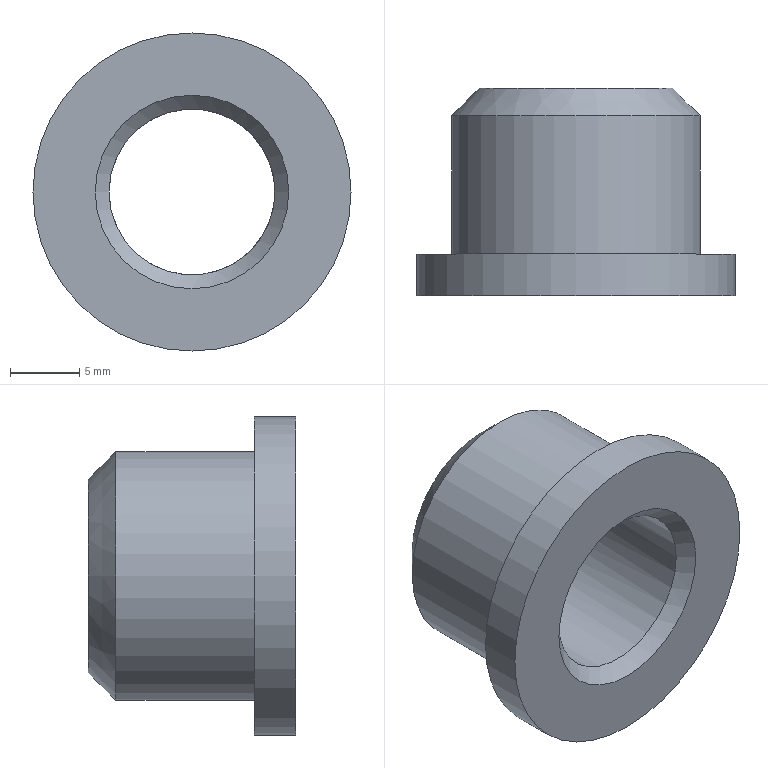Component | NX | LOCATING_BUSH | 1 solid | 8 faces | box 23 x 15 x 23 mm | volume 2479 mm3 | cylinder 3 | plane 3 | cone 2 | commonest cylinder face diameters 12 x1 18 x1 23 x1
STEP:
#1=CARTESIAN_POINT('',(0.,0.,0.));
#2=DIRECTION('',(0.,0.,1.));
#3=DIRECTION('',(1.,0.,0.));
#4=AXIS2_PLACEMENT_3D('',#1,#2,#3);
#5=CARTESIAN_POINT('',(-23.,5.,45.));
#6=VERTEX_POINT('',#5);
#7=CARTESIAN_POINT('',(-11.,5.,45.));
#8=VERTEX_POINT('',#7);
#9=CARTESIAN_POINT('',(-17.,5.,45.));
#10=DIRECTION('',(0.,-1.,0.));
#11=DIRECTION('',(1.,0.,0.));
#12=AXIS2_PLACEMENT_3D('',#9,#10,#11);
#13=CIRCLE('',#12,6.);
#14=CARTESIAN_POINT('',(-17.,19.,45.));
#15=DIRECTION('',(0.,1.,0.));
#16=DIRECTION('',(-1.,0.,0.));
#17=AXIS2_PLACEMENT_3D('',#14,#15,#16);
#18=CYLINDRICAL_SURFACE('',#17,6.);
#19=CARTESIAN_POINT('',(9.425,-14.));
#20=DIRECTION('',(-1.,0.));
#21=VECTOR('',#20,1.);
#22=LINE('',#19,#21);
#23=(GEOMETRIC_REPRESENTATION_CONTEXT(2)PARAMETRIC_REPRESENTATION_CONTEXT()REPRESENTATION_CONTEXT('',''));
#24=DEFINITIONAL_REPRESENTATION('',(#22),#23);
#25=PCURVE('',#18,#24);
#26=CARTESIAN_POINT('',(-17.,4.,45.));
#27=DIRECTION('',(0.,-1.,0.));
#28=DIRECTION('',(1.,0.,0.));
#29=AXIS2_PLACEMENT_3D('',#26,#27,#28);
#30=CONICAL_SURFACE('',#29,7.,0.7854);
#31=CARTESIAN_POINT('',(0.,-1.));
#32=DIRECTION('',(1.,0.));
#33=VECTOR('',#32,1.);
#34=LINE('',#31,#33);
#35=(GEOMETRIC_REPRESENTATION_CONTEXT(2)PARAMETRIC_REPRESENTATION_CONTEXT()REPRESENTATION_CONTEXT('',''));
#36=DEFINITIONAL_REPRESENTATION('',(#34),#35);
#37=PCURVE('',#30,#36);
#38=SURFACE_CURVE('',#13,(#25,#37),.PCURVE_S1.);
#39=EDGE_CURVE('',#6,#8,#38,.T.);
#40=ORIENTED_EDGE('',*,*,#39,.F.);
#41=CARTESIAN_POINT('',(-23.,19.,45.));
#42=VERTEX_POINT('',#41);
#43=CARTESIAN_POINT('',(-23.,5.,45.));
#44=CARTESIAN_POINT('',(-23.,19.,45.));
#45=B_SPLINE_CURVE_WITH_KNOTS('',1,(#43,#44),.UNSPECIFIED.,.F.,.F.,(2,2),(-14.,0.),.PIECEWISE_BEZIER_KNOTS.);
#46=CARTESIAN_POINT('',(6.283,0.));
#47=DIRECTION('',(0.,1.));
#48=VECTOR('',#47,1.);
#49=LINE('',#46,#48);
#50=(GEOMETRIC_REPRESENTATION_CONTEXT(2)PARAMETRIC_REPRESENTATION_CONTEXT()REPRESENTATION_CONTEXT('',''));
#51=DEFINITIONAL_REPRESENTATION('',(#49),#50);
#52=PCURVE('',#18,#51);
#53=CARTESIAN_POINT('',(0.,0.));
#54=DIRECTION('',(0.,1.));
#55=VECTOR('',#54,1.);
#56=LINE('',#53,#55);
#57=(GEOMETRIC_REPRESENTATION_CONTEXT(2)PARAMETRIC_REPRESENTATION_CONTEXT()REPRESENTATION_CONTEXT('',''));
#58=DEFINITIONAL_REPRESENTATION('',(#56),#57);
#59=PCURVE('',#18,#58);
#60=SEAM_CURVE('',#45,(#52,#59),.PCURVE_S1.);
#61=EDGE_CURVE('',#6,#42,#60,.T.);
#62=ORIENTED_EDGE('',*,*,#61,.T.);
#63=CARTESIAN_POINT('',(-17.,19.,45.));
#64=DIRECTION('',(0.,1.,0.));
#65=DIRECTION('',(-1.,0.,0.));
#66=AXIS2_PLACEMENT_3D('',#63,#64,#65);
#67=CIRCLE('',#66,6.);
#68=CARTESIAN_POINT('',(0.,0.));
#69=DIRECTION('',(1.,0.));
#70=VECTOR('',#69,1.);
#71=LINE('',#68,#70);
#72=(GEOMETRIC_REPRESENTATION_CONTEXT(2)PARAMETRIC_REPRESENTATION_CONTEXT()REPRESENTATION_CONTEXT('',''));
#73=DEFINITIONAL_REPRESENTATION('',(#71),#72);
#74=PCURVE('',#18,#73);
#75=CARTESIAN_POINT('',(-11.,19.,45.));
#76=DIRECTION('',(0.,1.,0.));
#77=DIRECTION('',(-1.,0.,0.));
#78=AXIS2_PLACEMENT_3D('',#75,#76,#77);
#79=PLANE('',#78);
#80=CARTESIAN_POINT('',(6.,0.));
#81=DIRECTION('',(1.,0.));
#82=AXIS2_PLACEMENT_2D('',#80,#81);
#83=CIRCLE('',#82,6.);
#84=(GEOMETRIC_REPRESENTATION_CONTEXT(2)PARAMETRIC_REPRESENTATION_CONTEXT()REPRESENTATION_CONTEXT('',''));
#85=DEFINITIONAL_REPRESENTATION('',(#83),#84);
#86=PCURVE('',#79,#85);
#87=SURFACE_CURVE('',#67,(#74,#86),.PCURVE_S1.);
#88=EDGE_CURVE('',#42,#42,#87,.T.);
#89=ORIENTED_EDGE('',*,*,#88,.F.);
#90=ORIENTED_EDGE('',*,*,#61,.F.);
#91=CARTESIAN_POINT('',(-17.,5.,45.));
#92=DIRECTION('',(0.,-1.,0.));
#93=DIRECTION('',(1.,0.,0.));
#94=AXIS2_PLACEMENT_3D('',#91,#92,#93);
#95=CIRCLE('',#94,6.);
#96=CARTESIAN_POINT('',(3.142,-14.));
#97=DIRECTION('',(-1.,0.));
#98=VECTOR('',#97,1.);
#99=LINE('',#96,#98);
#100=(GEOMETRIC_REPRESENTATION_CONTEXT(2)PARAMETRIC_REPRESENTATION_CONTEXT()REPRESENTATION_CONTEXT('',''));
#101=DEFINITIONAL_REPRESENTATION('',(#99),#100);
#102=PCURVE('',#18,#101);
#103=CARTESIAN_POINT('',(0.,-1.));
#104=DIRECTION('',(1.,0.));
#105=VECTOR('',#104,1.);
#106=LINE('',#103,#105);
#107=(GEOMETRIC_REPRESENTATION_CONTEXT(2)PARAMETRIC_REPRESENTATION_CONTEXT()REPRESENTATION_CONTEXT('',''));
#108=DEFINITIONAL_REPRESENTATION('',(#106),#107);
#109=PCURVE('',#30,#108);
#110=SURFACE_CURVE('',#95,(#102,#109),.PCURVE_S1.);
#111=EDGE_CURVE('',#8,#6,#110,.T.);
#112=ORIENTED_EDGE('',*,*,#111,.F.);
#113=EDGE_LOOP('',(#40,#62,#89,#90,#112));
#114=FACE_BOUND('',#113,.F.);
#115=ADVANCED_FACE('',(#114),#18,.F.);
#116=CARTESIAN_POINT('',(-24.,19.,45.));
#117=VERTEX_POINT('',#116);
#118=CARTESIAN_POINT('',(-17.,19.,45.));
#119=DIRECTION('',(0.,1.,0.));
#120=DIRECTION('',(-1.,0.,0.));
#121=AXIS2_PLACEMENT_3D('',#118,#119,#120);
#122=CIRCLE('',#121,7.);
#123=CARTESIAN_POINT('',(6.,0.));
#124=DIRECTION('',(1.,0.));
#125=AXIS2_PLACEMENT_2D('',#123,#124);
#126=CIRCLE('',#125,7.);
#127=(GEOMETRIC_REPRESENTATION_CONTEXT(2)PARAMETRIC_REPRESENTATION_CONTEXT()REPRESENTATION_CONTEXT('',''));
#128=DEFINITIONAL_REPRESENTATION('',(#126),#127);
#129=PCURVE('',#79,#128);
#130=CARTESIAN_POINT('',(-17.,19.,45.));
#131=DIRECTION('',(0.,-1.,0.));
#132=DIRECTION('',(1.,0.,0.));
#133=AXIS2_PLACEMENT_3D('',#130,#131,#132);
#134=CONICAL_SURFACE('',#133,7.,0.7854);
#135=CARTESIAN_POINT('',(9.425,0.));
#136=DIRECTION('',(-1.,0.));
#137=VECTOR('',#136,1.);
#138=LINE('',#135,#137);
#139=(GEOMETRIC_REPRESENTATION_CONTEXT(2)PARAMETRIC_REPRESENTATION_CONTEXT()REPRESENTATION_CONTEXT('',''));
#140=DEFINITIONAL_REPRESENTATION('',(#138),#139);
#141=PCURVE('',#134,#140);
#142=SURFACE_CURVE('',#122,(#129,#141),.PCURVE_S1.);
#143=EDGE_CURVE('',#117,#117,#142,.T.);
#144=ORIENTED_EDGE('',*,*,#143,.T.);
#145=EDGE_LOOP('',(#144));
#146=FACE_BOUND('',#145,.T.);
#147=ORIENTED_EDGE('',*,*,#88,.F.);
#148=EDGE_LOOP('',(#147));
#149=FACE_BOUND('',#148,.T.);
#150=ADVANCED_FACE('',(#146,#149),#79,.T.);
#151=CARTESIAN_POINT('',(-26.,17.,45.));
#152=VERTEX_POINT('',#151);
#153=CARTESIAN_POINT('',(-17.,17.,45.));
#154=DIRECTION('',(0.,-1.,0.));
#155=DIRECTION('',(-1.,0.,0.));
#156=AXIS2_PLACEMENT_3D('',#153,#154,#155);
#157=CIRCLE('',#156,9.);
#158=CARTESIAN_POINT('',(-17.,19.,45.));
#159=DIRECTION('',(0.,1.,0.));
#160=DIRECTION('',(-1.,0.,0.));
#161=AXIS2_PLACEMENT_3D('',#158,#159,#160);
#162=CYLINDRICAL_SURFACE('',#161,9.);
#163=CARTESIAN_POINT('',(6.283,-2.));
#164=DIRECTION('',(-1.,0.));
#165=VECTOR('',#164,1.);
#166=LINE('',#163,#165);
#167=(GEOMETRIC_REPRESENTATION_CONTEXT(2)PARAMETRIC_REPRESENTATION_CONTEXT()REPRESENTATION_CONTEXT('',''));
#168=DEFINITIONAL_REPRESENTATION('',(#166),#167);
#169=PCURVE('',#162,#168);
#170=CARTESIAN_POINT('',(3.142,2.));
#171=DIRECTION('',(1.,0.));
#172=VECTOR('',#171,1.);
#173=LINE('',#170,#172);
#174=(GEOMETRIC_REPRESENTATION_CONTEXT(2)PARAMETRIC_REPRESENTATION_CONTEXT()REPRESENTATION_CONTEXT('',''));
#175=DEFINITIONAL_REPRESENTATION('',(#173),#174);
#176=PCURVE('',#134,#175);
#177=SURFACE_CURVE('',#157,(#169,#176),.PCURVE_S1.);
#178=EDGE_CURVE('',#152,#152,#177,.T.);
#179=ORIENTED_EDGE('',*,*,#178,.T.);
#180=CARTESIAN_POINT('',(-26.,7.,45.));
#181=VERTEX_POINT('',#180);
#182=CARTESIAN_POINT('',(-26.,7.,45.));
#183=CARTESIAN_POINT('',(-26.,17.,45.));
#184=B_SPLINE_CURVE_WITH_KNOTS('',1,(#182,#183),.UNSPECIFIED.,.F.,.F.,(2,2),(-12.,-2.),.PIECEWISE_BEZIER_KNOTS.);
#185=CARTESIAN_POINT('',(0.,0.));
#186=DIRECTION('',(0.,1.));
#187=VECTOR('',#186,1.);
#188=LINE('',#185,#187);
#189=(GEOMETRIC_REPRESENTATION_CONTEXT(2)PARAMETRIC_REPRESENTATION_CONTEXT()REPRESENTATION_CONTEXT('',''));
#190=DEFINITIONAL_REPRESENTATION('',(#188),#189);
#191=PCURVE('',#162,#190);
#192=CARTESIAN_POINT('',(6.283,0.));
#193=DIRECTION('',(0.,1.));
#194=VECTOR('',#193,1.);
#195=LINE('',#192,#194);
#196=(GEOMETRIC_REPRESENTATION_CONTEXT(2)PARAMETRIC_REPRESENTATION_CONTEXT()REPRESENTATION_CONTEXT('',''));
#197=DEFINITIONAL_REPRESENTATION('',(#195),#196);
#198=PCURVE('',#162,#197);
#199=SEAM_CURVE('',#184,(#191,#198),.PCURVE_S1.);
#200=EDGE_CURVE('',#181,#152,#199,.T.);
#201=ORIENTED_EDGE('',*,*,#200,.F.);
#202=CARTESIAN_POINT('',(-17.,7.,45.));
#203=DIRECTION('',(0.,1.,0.));
#204=DIRECTION('',(-1.,0.,0.));
#205=AXIS2_PLACEMENT_3D('',#202,#203,#204);
#206=CIRCLE('',#205,9.);
#207=CARTESIAN_POINT('',(0.,-12.));
#208=DIRECTION('',(1.,0.));
#209=VECTOR('',#208,1.);
#210=LINE('',#207,#209);
#211=(GEOMETRIC_REPRESENTATION_CONTEXT(2)PARAMETRIC_REPRESENTATION_CONTEXT()REPRESENTATION_CONTEXT('',''));
#212=DEFINITIONAL_REPRESENTATION('',(#210),#211);
#213=PCURVE('',#162,#212);
#214=CARTESIAN_POINT('',(-8.,7.,45.));
#215=DIRECTION('',(0.,1.,0.));
#216=DIRECTION('',(-1.,0.,0.));
#217=AXIS2_PLACEMENT_3D('',#214,#215,#216);
#218=PLANE('',#217);
#219=CARTESIAN_POINT('',(9.,0.));
#220=DIRECTION('',(1.,0.));
#221=AXIS2_PLACEMENT_2D('',#219,#220);
#222=CIRCLE('',#221,9.);
#223=(GEOMETRIC_REPRESENTATION_CONTEXT(2)PARAMETRIC_REPRESENTATION_CONTEXT()REPRESENTATION_CONTEXT('',''));
#224=DEFINITIONAL_REPRESENTATION('',(#222),#223);
#225=PCURVE('',#218,#224);
#226=SURFACE_CURVE('',#206,(#213,#225),.PCURVE_S1.);
#227=EDGE_CURVE('',#181,#181,#226,.T.);
#228=ORIENTED_EDGE('',*,*,#227,.T.);
#229=ORIENTED_EDGE('',*,*,#200,.T.);
#230=EDGE_LOOP('',(#179,#201,#228,#229));
#231=FACE_BOUND('',#230,.T.);
#232=ADVANCED_FACE('',(#231),#162,.T.);
#233=CARTESIAN_POINT('',(-28.5,7.,45.));
#234=VERTEX_POINT('',#233);
#235=CARTESIAN_POINT('',(-17.,7.,45.));
#236=DIRECTION('',(0.,1.,0.));
#237=DIRECTION('',(-1.,0.,0.));
#238=AXIS2_PLACEMENT_3D('',#235,#236,#237);
#239=CIRCLE('',#238,11.5);
#240=CARTESIAN_POINT('',(9.,0.));
#241=DIRECTION('',(1.,0.));
#242=AXIS2_PLACEMENT_2D('',#240,#241);
#243=CIRCLE('',#242,11.5);
#244=(GEOMETRIC_REPRESENTATION_CONTEXT(2)PARAMETRIC_REPRESENTATION_CONTEXT()REPRESENTATION_CONTEXT('',''));
#245=DEFINITIONAL_REPRESENTATION('',(#243),#244);
#246=PCURVE('',#218,#245);
#247=CARTESIAN_POINT('',(-17.,19.,45.));
#248=DIRECTION('',(0.,1.,0.));
#249=DIRECTION('',(-1.,0.,0.));
#250=AXIS2_PLACEMENT_3D('',#247,#248,#249);
#251=CYLINDRICAL_SURFACE('',#250,11.5);
#252=CARTESIAN_POINT('',(0.,-12.));
#253=DIRECTION('',(1.,0.));
#254=VECTOR('',#253,1.);
#255=LINE('',#252,#254);
#256=(GEOMETRIC_REPRESENTATION_CONTEXT(2)PARAMETRIC_REPRESENTATION_CONTEXT()REPRESENTATION_CONTEXT('',''));
#257=DEFINITIONAL_REPRESENTATION('',(#255),#256);
#258=PCURVE('',#251,#257);
#259=SURFACE_CURVE('',#239,(#246,#258),.PCURVE_S1.);
#260=EDGE_CURVE('',#234,#234,#259,.T.);
#261=ORIENTED_EDGE('',*,*,#260,.T.);
#262=EDGE_LOOP('',(#261));
#263=FACE_BOUND('',#262,.T.);
#264=ORIENTED_EDGE('',*,*,#227,.F.);
#265=EDGE_LOOP('',(#264));
#266=FACE_BOUND('',#265,.T.);
#267=ADVANCED_FACE('',(#263,#266),#218,.T.);
#268=CARTESIAN_POINT('',(-28.5,4.,45.));
#269=VERTEX_POINT('',#268);
#270=CARTESIAN_POINT('',(-17.,4.,45.));
#271=DIRECTION('',(0.,1.,0.));
#272=DIRECTION('',(-1.,0.,0.));
#273=AXIS2_PLACEMENT_3D('',#270,#271,#272);
#274=CIRCLE('',#273,11.5);
#275=CARTESIAN_POINT('',(0.,-15.));
#276=DIRECTION('',(1.,0.));
#277=VECTOR('',#276,1.);
#278=LINE('',#275,#277);
#279=(GEOMETRIC_REPRESENTATION_CONTEXT(2)PARAMETRIC_REPRESENTATION_CONTEXT()REPRESENTATION_CONTEXT('',''));
#280=DEFINITIONAL_REPRESENTATION('',(#278),#279);
#281=PCURVE('',#251,#280);
#282=CARTESIAN_POINT('',(-5.5,4.,45.));
#283=DIRECTION('',(0.,-1.,0.));
#284=DIRECTION('',(1.,0.,0.));
#285=AXIS2_PLACEMENT_3D('',#282,#283,#284);
#286=PLANE('',#285);
#287=CARTESIAN_POINT('',(-23.,0.));
#288=CARTESIAN_POINT('',(-23.,19.919));
#289=CARTESIAN_POINT('',(-5.75,9.959));
#290=CARTESIAN_POINT('',(11.5,0.));
#291=CARTESIAN_POINT('',(-5.75,-9.959));
#292=CARTESIAN_POINT('',(-23.,-19.919));
#293=CARTESIAN_POINT('',(-23.,0.));
#294=(BOUNDED_CURVE()B_SPLINE_CURVE(2,(#287,#288,#289,#290,#291,#292,#293),.UNSPECIFIED.,.T.,.F.)B_SPLINE_CURVE_WITH_KNOTS((1,2,2,2,2,1),(-2.094,0.,2.094,4.189,6.283,8.378),.UNSPECIFIED.)CURVE()GEOMETRIC_REPRESENTATION_ITEM()RATIONAL_B_SPLINE_CURVE((1.,0.5,1.,0.5,1.,0.5,1.))REPRESENTATION_ITEM(''));
#295=(GEOMETRIC_REPRESENTATION_CONTEXT(2)PARAMETRIC_REPRESENTATION_CONTEXT()REPRESENTATION_CONTEXT('',''));
#296=DEFINITIONAL_REPRESENTATION('',(#294),#295);
#297=PCURVE('',#286,#296);
#298=SURFACE_CURVE('',#274,(#281,#297),.PCURVE_S1.);
#299=EDGE_CURVE('',#269,#269,#298,.T.);
#300=ORIENTED_EDGE('',*,*,#299,.T.);
#301=CARTESIAN_POINT('',(-28.5,4.,45.));
#302=CARTESIAN_POINT('',(-28.5,7.,45.));
#303=B_SPLINE_CURVE_WITH_KNOTS('',1,(#301,#302),.UNSPECIFIED.,.F.,.F.,(2,2),(-15.,-12.),.PIECEWISE_BEZIER_KNOTS.);
#304=CARTESIAN_POINT('',(6.283,0.));
#305=DIRECTION('',(0.,1.));
#306=VECTOR('',#305,1.);
#307=LINE('',#304,#306);
#308=(GEOMETRIC_REPRESENTATION_CONTEXT(2)PARAMETRIC_REPRESENTATION_CONTEXT()REPRESENTATION_CONTEXT('',''));
#309=DEFINITIONAL_REPRESENTATION('',(#307),#308);
#310=PCURVE('',#251,#309);
#311=CARTESIAN_POINT('',(0.,0.));
#312=DIRECTION('',(0.,1.));
#313=VECTOR('',#312,1.);
#314=LINE('',#311,#313);
#315=(GEOMETRIC_REPRESENTATION_CONTEXT(2)PARAMETRIC_REPRESENTATION_CONTEXT()REPRESENTATION_CONTEXT('',''));
#316=DEFINITIONAL_REPRESENTATION('',(#314),#315);
#317=PCURVE('',#251,#316);
#318=SEAM_CURVE('',#303,(#310,#317),.PCURVE_S1.);
#319=EDGE_CURVE('',#269,#234,#318,.T.);
#320=ORIENTED_EDGE('',*,*,#319,.T.);
#321=ORIENTED_EDGE('',*,*,#260,.F.);
#322=ORIENTED_EDGE('',*,*,#319,.F.);
#323=EDGE_LOOP('',(#300,#320,#321,#322));
#324=FACE_BOUND('',#323,.T.);
#325=ADVANCED_FACE('',(#324),#251,.T.);
#326=CARTESIAN_POINT('',(-10.,4.,45.));
#327=VERTEX_POINT('',#326);
#328=CARTESIAN_POINT('',(-17.,4.,45.));
#329=DIRECTION('',(0.,1.,0.));
#330=DIRECTION('',(1.,0.,0.));
#331=AXIS2_PLACEMENT_3D('',#328,#329,#330);
#332=CIRCLE('',#331,7.);
#333=CARTESIAN_POINT('',(-4.5,0.));
#334=CARTESIAN_POINT('',(-4.5,-12.124));
#335=CARTESIAN_POINT('',(-15.,-6.062));
#336=CARTESIAN_POINT('',(-25.5,-0.));
#337=CARTESIAN_POINT('',(-15.,6.062));
#338=CARTESIAN_POINT('',(-4.5,12.124));
#339=CARTESIAN_POINT('',(-4.5,0.));
#340=(BOUNDED_CURVE()B_SPLINE_CURVE(2,(#333,#334,#335,#336,#337,#338,#339),.UNSPECIFIED.,.T.,.F.)B_SPLINE_CURVE_WITH_KNOTS((1,2,2,2,2,1),(-2.094,0.,2.094,4.189,6.283,8.378),.UNSPECIFIED.)CURVE()GEOMETRIC_REPRESENTATION_ITEM()RATIONAL_B_SPLINE_CURVE((1.,0.5,1.,0.5,1.,0.5,1.))REPRESENTATION_ITEM(''));
#341=(GEOMETRIC_REPRESENTATION_CONTEXT(2)PARAMETRIC_REPRESENTATION_CONTEXT()REPRESENTATION_CONTEXT('',''));
#342=DEFINITIONAL_REPRESENTATION('',(#340),#341);
#343=PCURVE('',#286,#342);
#344=CARTESIAN_POINT('',(6.283,0.));
#345=DIRECTION('',(-1.,0.));
#346=VECTOR('',#345,1.);
#347=LINE('',#344,#346);
#348=(GEOMETRIC_REPRESENTATION_CONTEXT(2)PARAMETRIC_REPRESENTATION_CONTEXT()REPRESENTATION_CONTEXT('',''));
#349=DEFINITIONAL_REPRESENTATION('',(#347),#348);
#350=PCURVE('',#30,#349);
#351=SURFACE_CURVE('',#332,(#343,#350),.PCURVE_S1.);
#352=EDGE_CURVE('',#327,#327,#351,.T.);
#353=ORIENTED_EDGE('',*,*,#352,.T.);
#354=EDGE_LOOP('',(#353));
#355=FACE_BOUND('',#354,.T.);
#356=ORIENTED_EDGE('',*,*,#299,.F.);
#357=EDGE_LOOP('',(#356));
#358=FACE_BOUND('',#357,.T.);
#359=ADVANCED_FACE('',(#355,#358),#286,.T.);
#360=ORIENTED_EDGE('',*,*,#178,.F.);
#361=CARTESIAN_POINT('',(-24.,19.,45.));
#362=CARTESIAN_POINT('',(-26.,17.,45.));
#363=B_SPLINE_CURVE_WITH_KNOTS('',1,(#361,#362),.UNSPECIFIED.,.F.,.F.,(2,2),(0.,2.828),.PIECEWISE_BEZIER_KNOTS.);
#364=CARTESIAN_POINT('',(3.142,0.));
#365=DIRECTION('',(0.,1.));
#366=VECTOR('',#365,1.);
#367=LINE('',#364,#366);
#368=(GEOMETRIC_REPRESENTATION_CONTEXT(2)PARAMETRIC_REPRESENTATION_CONTEXT()REPRESENTATION_CONTEXT('',''));
#369=DEFINITIONAL_REPRESENTATION('',(#367),#368);
#370=PCURVE('',#134,#369);
#371=CARTESIAN_POINT('',(9.425,0.));
#372=DIRECTION('',(0.,1.));
#373=VECTOR('',#372,1.);
#374=LINE('',#371,#373);
#375=(GEOMETRIC_REPRESENTATION_CONTEXT(2)PARAMETRIC_REPRESENTATION_CONTEXT()REPRESENTATION_CONTEXT('',''));
#376=DEFINITIONAL_REPRESENTATION('',(#374),#375);
#377=PCURVE('',#134,#376);
#378=SEAM_CURVE('',#363,(#370,#377),.PCURVE_S1.);
#379=EDGE_CURVE('',#117,#152,#378,.T.);
#380=ORIENTED_EDGE('',*,*,#379,.F.);
#381=ORIENTED_EDGE('',*,*,#143,.F.);
#382=ORIENTED_EDGE('',*,*,#379,.T.);
#383=EDGE_LOOP('',(#360,#380,#381,#382));
#384=FACE_BOUND('',#383,.T.);
#385=ADVANCED_FACE('',(#384),#134,.T.);
#386=ORIENTED_EDGE('',*,*,#39,.T.);
#387=CARTESIAN_POINT('',(-11.,5.,45.));
#388=CARTESIAN_POINT('',(-10.,4.,45.));
#389=B_SPLINE_CURVE_WITH_KNOTS('',1,(#387,#388),.UNSPECIFIED.,.F.,.F.,(2,2),(-1.414,0.),.PIECEWISE_BEZIER_KNOTS.);
#390=CARTESIAN_POINT('',(6.283,0.));
#391=DIRECTION('',(0.,1.));
#392=VECTOR('',#391,1.);
#393=LINE('',#390,#392);
#394=(GEOMETRIC_REPRESENTATION_CONTEXT(2)PARAMETRIC_REPRESENTATION_CONTEXT()REPRESENTATION_CONTEXT('',''));
#395=DEFINITIONAL_REPRESENTATION('',(#393),#394);
#396=PCURVE('',#30,#395);
#397=CARTESIAN_POINT('',(0.,0.));
#398=DIRECTION('',(0.,1.));
#399=VECTOR('',#398,1.);
#400=LINE('',#397,#399);
#401=(GEOMETRIC_REPRESENTATION_CONTEXT(2)PARAMETRIC_REPRESENTATION_CONTEXT()REPRESENTATION_CONTEXT('',''));
#402=DEFINITIONAL_REPRESENTATION('',(#400),#401);
#403=PCURVE('',#30,#402);
#404=SEAM_CURVE('',#389,(#396,#403),.PCURVE_S1.);
#405=EDGE_CURVE('',#8,#327,#404,.T.);
#406=ORIENTED_EDGE('',*,*,#405,.T.);
#407=ORIENTED_EDGE('',*,*,#352,.T.);
#408=ORIENTED_EDGE('',*,*,#405,.F.);
#409=ORIENTED_EDGE('',*,*,#111,.T.);
#410=EDGE_LOOP('',(#386,#406,#407,#408,#409));
#411=FACE_BOUND('',#410,.F.);
#412=ADVANCED_FACE('',(#411),#30,.F.);
#413=CLOSED_SHELL('',(#115,#150,#232,#267,#325,#359,#385,#412));
#414=MANIFOLD_SOLID_BREP('',#413);
#415=(LENGTH_UNIT()NAMED_UNIT(*)SI_UNIT(.MILLI.,.METRE.));
#416=UNCERTAINTY_MEASURE_WITH_UNIT(LENGTH_MEASURE(0.00001),#415,'','');
#417=(NAMED_UNIT(*)PLANE_ANGLE_UNIT()SI_UNIT($,.RADIAN.));
#418=(NAMED_UNIT(*)SI_UNIT($,.STERADIAN.)SOLID_ANGLE_UNIT());
#419=(GEOMETRIC_REPRESENTATION_CONTEXT(3)GLOBAL_UNCERTAINTY_ASSIGNED_CONTEXT((#416))GLOBAL_UNIT_ASSIGNED_CONTEXT((#415,#417,#418))REPRESENTATION_CONTEXT('',''));
#420=ADVANCED_BREP_SHAPE_REPRESENTATION('',(#4,#414),#419);